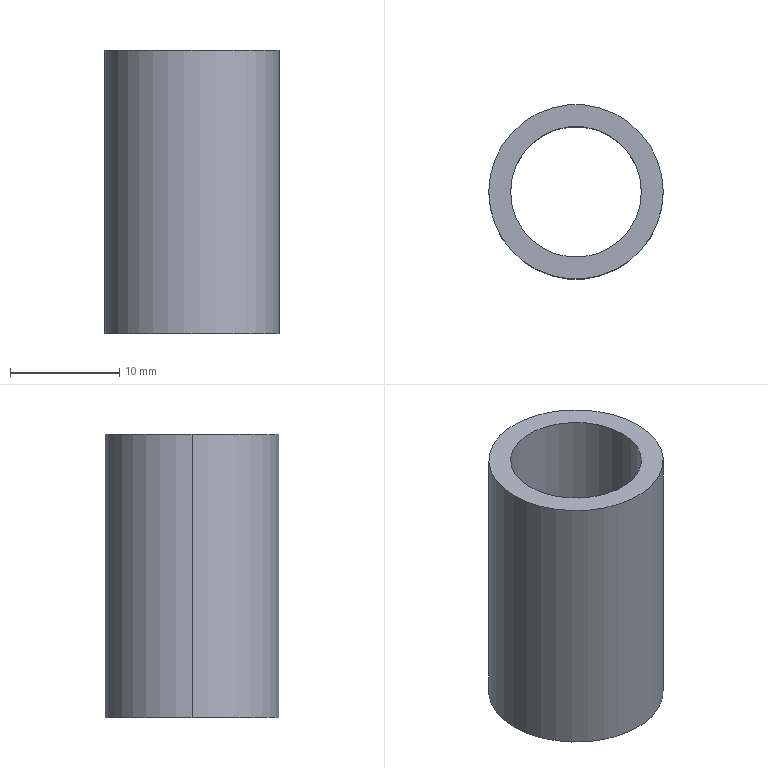Component | SolidWorks | BSH3-03-08CopperRing-1 | 1 solid | 6 faces | box 16 x 16 x 26 mm | volume 2287 mm3 | cylinder 4 | plane 2 | commonest cylinder face diameters 12 x2 16 x2
build123d program:
from build123d import *

# Parameters (mm, degrees)
SKETCH1_R      = 8
SKETCH1_R_2    = 6
EXTRUDE1_DEPTH = 26


with BuildPart() as part:
    # Sketch1 → Extrude1 (new body)
    with BuildSketch(Plane.XY):
        with Locations(Location((0, 0, 0), (0, 0, 180))):
            Circle(SKETCH1_R)
        with Locations(Location((0, 0, 0), (0, 0, 180))):
            Circle(SKETCH1_R_2, mode=Mode.SUBTRACT)
    extrude(amount=EXTRUDE1_DEPTH)


solid = part.part

# Placed as in the assembly
solid = solid.moved(Location((-60.871, 27.262, -25.939), (0, 0, 0)))
STEP:
#1=CARTESIAN_POINT('',(-2.633,1.073,0.002394));
#2=VERTEX_POINT('',#1);
#3=CARTESIAN_POINT('',(-2.16,1.073,0.002394));
#4=VERTEX_POINT('',#3);
#5=CARTESIAN_POINT('',(-2.396,1.073,0.002394));
#6=DIRECTION('',(0.,0.,1.));
#7=DIRECTION('',(1.,0.,0.));
#8=AXIS2_PLACEMENT_3D('',#5,#6,#7);
#9=CIRCLE('',#8,0.2362);
#10=EDGE_CURVE('',#2,#4,#9,.T.);
#11=ORIENTED_EDGE('',*,*,#10,.T.);
#12=CARTESIAN_POINT('',(-2.16,1.073,-1.021));
#13=VERTEX_POINT('',#12);
#14=CARTESIAN_POINT('',(-2.16,1.073,0.002394));
#15=DIRECTION('',(0.,0.,-1.));
#16=VECTOR('',#15,39.37);
#17=LINE('',#14,#16);
#18=EDGE_CURVE('',#4,#13,#17,.T.);
#19=ORIENTED_EDGE('',*,*,#18,.T.);
#20=CARTESIAN_POINT('',(-2.633,1.073,-1.021));
#21=VERTEX_POINT('',#20);
#22=CARTESIAN_POINT('',(-2.396,1.073,-1.021));
#23=DIRECTION('',(0.,0.,1.));
#24=DIRECTION('',(1.,0.,0.));
#25=AXIS2_PLACEMENT_3D('',#22,#23,#24);
#26=CIRCLE('',#25,0.2362);
#27=EDGE_CURVE('',#21,#13,#26,.T.);
#28=ORIENTED_EDGE('',*,*,#27,.F.);
#29=CARTESIAN_POINT('',(-2.633,1.073,0.002394));
#30=DIRECTION('',(0.,0.,-1.));
#31=VECTOR('',#30,39.37);
#32=LINE('',#29,#31);
#33=EDGE_CURVE('',#2,#21,#32,.T.);
#34=ORIENTED_EDGE('',*,*,#33,.F.);
#35=EDGE_LOOP('',(#11,#19,#28,#34));
#36=FACE_OUTER_BOUND('',#35,.T.);
#37=CARTESIAN_POINT('',(-2.396,1.073,0.002394));
#38=DIRECTION('',(0.,0.,-1.));
#39=DIRECTION('',(-1.,0.,0.));
#40=AXIS2_PLACEMENT_3D('',#37,#38,#39);
#41=CYLINDRICAL_SURFACE('',#40,0.2362);
#42=ADVANCED_FACE('',(#36),#41,.F.);
#43=CARTESIAN_POINT('',(-2.082,1.073,0.002394));
#44=VERTEX_POINT('',#43);
#45=CARTESIAN_POINT('',(-2.711,1.073,0.002394));
#46=VERTEX_POINT('',#45);
#47=CARTESIAN_POINT('',(-2.396,1.073,0.002394));
#48=DIRECTION('',(0.,0.,1.));
#49=DIRECTION('',(1.,0.,0.));
#50=AXIS2_PLACEMENT_3D('',#47,#48,#49);
#51=CIRCLE('',#50,0.315);
#52=EDGE_CURVE('',#44,#46,#51,.T.);
#53=ORIENTED_EDGE('',*,*,#52,.F.);
#54=CARTESIAN_POINT('',(-2.082,1.073,-1.021));
#55=VERTEX_POINT('',#54);
#56=CARTESIAN_POINT('',(-2.082,1.073,0.002394));
#57=DIRECTION('',(0.,0.,-1.));
#58=VECTOR('',#57,39.37);
#59=LINE('',#56,#58);
#60=EDGE_CURVE('',#44,#55,#59,.T.);
#61=ORIENTED_EDGE('',*,*,#60,.T.);
#62=CARTESIAN_POINT('',(-2.711,1.073,-1.021));
#63=VERTEX_POINT('',#62);
#64=CARTESIAN_POINT('',(-2.396,1.073,-1.021));
#65=DIRECTION('',(0.,0.,1.));
#66=DIRECTION('',(1.,0.,0.));
#67=AXIS2_PLACEMENT_3D('',#64,#65,#66);
#68=CIRCLE('',#67,0.315);
#69=EDGE_CURVE('',#55,#63,#68,.T.);
#70=ORIENTED_EDGE('',*,*,#69,.T.);
#71=CARTESIAN_POINT('',(-2.711,1.073,0.002394));
#72=DIRECTION('',(0.,0.,-1.));
#73=VECTOR('',#72,39.37);
#74=LINE('',#71,#73);
#75=EDGE_CURVE('',#46,#63,#74,.T.);
#76=ORIENTED_EDGE('',*,*,#75,.F.);
#77=EDGE_LOOP('',(#53,#61,#70,#76));
#78=FACE_OUTER_BOUND('',#77,.T.);
#79=CARTESIAN_POINT('',(-2.396,1.073,0.002394));
#80=DIRECTION('',(0.,0.,-1.));
#81=DIRECTION('',(-1.,0.,0.));
#82=AXIS2_PLACEMENT_3D('',#79,#80,#81);
#83=CYLINDRICAL_SURFACE('',#82,0.315);
#84=ADVANCED_FACE('',(#78),#83,.T.);
#85=CARTESIAN_POINT('',(-2.396,1.073,0.002394));
#86=DIRECTION('',(0.,0.,1.));
#87=DIRECTION('',(1.,0.,0.));
#88=AXIS2_PLACEMENT_3D('',#85,#86,#87);
#89=CIRCLE('',#88,0.315);
#90=EDGE_CURVE('',#46,#44,#89,.T.);
#91=ORIENTED_EDGE('',*,*,#90,.T.);
#92=ORIENTED_EDGE('',*,*,#52,.T.);
#93=EDGE_LOOP('',(#91,#92));
#94=FACE_OUTER_BOUND('',#93,.T.);
#95=ORIENTED_EDGE('',*,*,#10,.F.);
#96=CARTESIAN_POINT('',(-2.396,1.073,0.002394));
#97=DIRECTION('',(0.,0.,1.));
#98=DIRECTION('',(1.,0.,0.));
#99=AXIS2_PLACEMENT_3D('',#96,#97,#98);
#100=CIRCLE('',#99,0.2362);
#101=EDGE_CURVE('',#4,#2,#100,.T.);
#102=ORIENTED_EDGE('',*,*,#101,.F.);
#103=EDGE_LOOP('',(#95,#102));
#104=FACE_BOUND('',#103,.T.);
#105=CARTESIAN_POINT('',(-2.396,1.073,0.002394));
#106=DIRECTION('',(0.,0.,1.));
#107=DIRECTION('',(1.,0.,0.));
#108=AXIS2_PLACEMENT_3D('',#105,#106,#107);
#109=PLANE('',#108);
#110=ADVANCED_FACE('',(#94,#104),#109,.T.);
#111=CARTESIAN_POINT('',(-2.396,1.073,-1.021));
#112=DIRECTION('',(0.,0.,1.));
#113=DIRECTION('',(1.,0.,0.));
#114=AXIS2_PLACEMENT_3D('',#111,#112,#113);
#115=CIRCLE('',#114,0.315);
#116=EDGE_CURVE('',#63,#55,#115,.T.);
#117=ORIENTED_EDGE('',*,*,#116,.F.);
#118=ORIENTED_EDGE('',*,*,#69,.F.);
#119=EDGE_LOOP('',(#117,#118));
#120=FACE_OUTER_BOUND('',#119,.T.);
#121=ORIENTED_EDGE('',*,*,#27,.T.);
#122=CARTESIAN_POINT('',(-2.396,1.073,-1.021));
#123=DIRECTION('',(0.,0.,1.));
#124=DIRECTION('',(1.,0.,0.));
#125=AXIS2_PLACEMENT_3D('',#122,#123,#124);
#126=CIRCLE('',#125,0.2362);
#127=EDGE_CURVE('',#13,#21,#126,.T.);
#128=ORIENTED_EDGE('',*,*,#127,.T.);
#129=EDGE_LOOP('',(#121,#128));
#130=FACE_BOUND('',#129,.T.);
#131=CARTESIAN_POINT('',(-2.396,1.073,-1.021));
#132=DIRECTION('',(0.,0.,1.));
#133=DIRECTION('',(1.,0.,0.));
#134=AXIS2_PLACEMENT_3D('',#131,#132,#133);
#135=PLANE('',#134);
#136=ADVANCED_FACE('',(#120,#130),#135,.F.);
#137=ORIENTED_EDGE('',*,*,#60,.F.);
#138=ORIENTED_EDGE('',*,*,#90,.F.);
#139=ORIENTED_EDGE('',*,*,#75,.T.);
#140=ORIENTED_EDGE('',*,*,#116,.T.);
#141=EDGE_LOOP('',(#137,#138,#139,#140));
#142=FACE_OUTER_BOUND('',#141,.T.);
#143=CARTESIAN_POINT('',(-2.396,1.073,0.002394));
#144=DIRECTION('',(0.,0.,-1.));
#145=DIRECTION('',(-1.,0.,0.));
#146=AXIS2_PLACEMENT_3D('',#143,#144,#145);
#147=CYLINDRICAL_SURFACE('',#146,0.315);
#148=ADVANCED_FACE('',(#142),#147,.T.);
#149=ORIENTED_EDGE('',*,*,#18,.F.);
#150=ORIENTED_EDGE('',*,*,#101,.T.);
#151=ORIENTED_EDGE('',*,*,#33,.T.);
#152=ORIENTED_EDGE('',*,*,#127,.F.);
#153=EDGE_LOOP('',(#149,#150,#151,#152));
#154=FACE_OUTER_BOUND('',#153,.T.);
#155=CARTESIAN_POINT('',(-2.396,1.073,0.002394));
#156=DIRECTION('',(0.,0.,-1.));
#157=DIRECTION('',(-1.,0.,0.));
#158=AXIS2_PLACEMENT_3D('',#155,#156,#157);
#159=CYLINDRICAL_SURFACE('',#158,0.2362);
#160=ADVANCED_FACE('',(#154),#159,.F.);
#161=CLOSED_SHELL('',(#42,#84,#110,#136,#148,#160));
#162=MANIFOLD_SOLID_BREP('',#161);
#163=CARTESIAN_POINT('',(0.,0.,0.));
#164=DIRECTION('',(0.,0.,1.));
#165=DIRECTION('',(1.,0.,0.));
#166=AXIS2_PLACEMENT_3D('',#163,#164,#165);
#167=(LENGTH_UNIT()NAMED_UNIT(*)SI_UNIT($,.METRE.));
#168=LENGTH_MEASURE_WITH_UNIT(LENGTH_MEASURE(0.0254),#167);
#169=DIMENSIONAL_EXPONENTS(1.,0.,0.,0.,0.,0.,0.);
#170=(CONVERSION_BASED_UNIT('',#168)LENGTH_UNIT()NAMED_UNIT(#169));
#171=UNCERTAINTY_MEASURE_WITH_UNIT(LENGTH_MEASURE(0.00001),#170,'','');
#172=(NAMED_UNIT(*)PLANE_ANGLE_UNIT()SI_UNIT($,.RADIAN.));
#173=(NAMED_UNIT(*)SI_UNIT($,.STERADIAN.)SOLID_ANGLE_UNIT());
#174=(GEOMETRIC_REPRESENTATION_CONTEXT(3)GLOBAL_UNCERTAINTY_ASSIGNED_CONTEXT((#171))GLOBAL_UNIT_ASSIGNED_CONTEXT((#170,#172,#173))REPRESENTATION_CONTEXT('',''));
#175=ADVANCED_BREP_SHAPE_REPRESENTATION('',(#162,#166),#174);
#176=COLOUR_RGB('',0.7922,0.8196,0.9333);
#177=FILL_AREA_STYLE_COLOUR('',#176);
#178=FILL_AREA_STYLE('',(#177));
#179=SURFACE_STYLE_FILL_AREA(#178);
#180=SURFACE_SIDE_STYLE('',(#179));
#181=SURFACE_STYLE_USAGE(.BOTH.,#180);
#182=PRESENTATION_STYLE_ASSIGNMENT((#181));
#183=STYLED_ITEM('',(#182),#162);
#184=(LENGTH_UNIT()NAMED_UNIT(*)SI_UNIT($,.METRE.));
#185=LENGTH_MEASURE_WITH_UNIT(LENGTH_MEASURE(0.0254),#184);
#186=DIMENSIONAL_EXPONENTS(1.,0.,0.,0.,0.,0.,0.);
#187=(CONVERSION_BASED_UNIT('',#185)LENGTH_UNIT()NAMED_UNIT(#186));
#188=UNCERTAINTY_MEASURE_WITH_UNIT(LENGTH_MEASURE(0.00001),#187,'','');
#189=(NAMED_UNIT(*)PLANE_ANGLE_UNIT()SI_UNIT($,.RADIAN.));
#190=(NAMED_UNIT(*)SI_UNIT($,.STERADIAN.)SOLID_ANGLE_UNIT());
#191=(GEOMETRIC_REPRESENTATION_CONTEXT(3)GLOBAL_UNCERTAINTY_ASSIGNED_CONTEXT((#188))GLOBAL_UNIT_ASSIGNED_CONTEXT((#187,#189,#190))REPRESENTATION_CONTEXT('',''));
#192=MECHANICAL_DESIGN_GEOMETRIC_PRESENTATION_REPRESENTATION('',(#183),#191);
#193=PRESENTATION_LAYER_ASSIGNMENT('','',(#183));